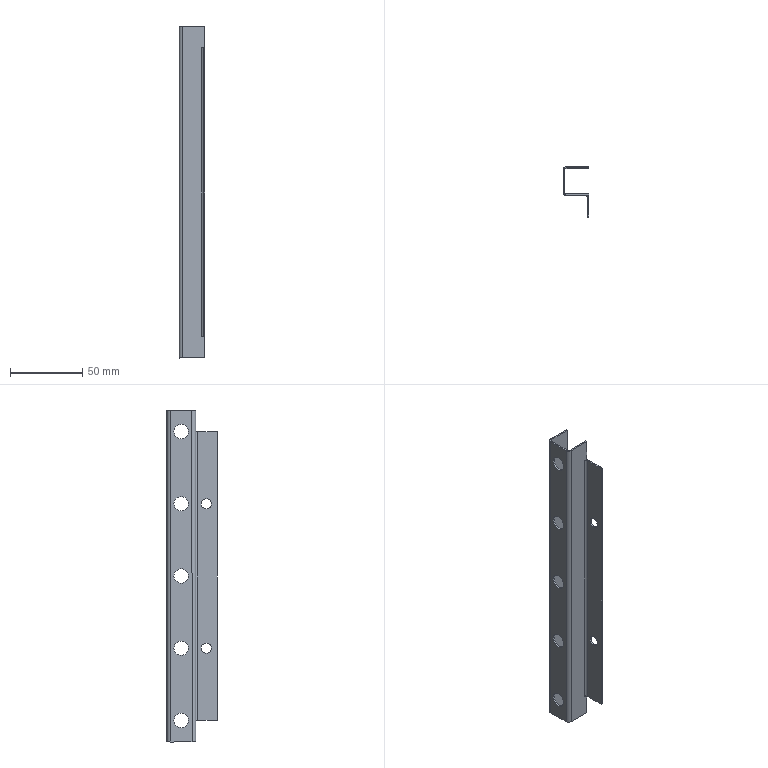Component | SolidWorks | RightFrontDoorAssembly-1_RightFrontDoorHorizontalStiffener06-02-2 | 1 solid | 48 faces | volume 14384 mm3 | plane 28 | cylinder 20 | commonest cylinder face diameters 10 x10 7 x4 5 x3 3 x3